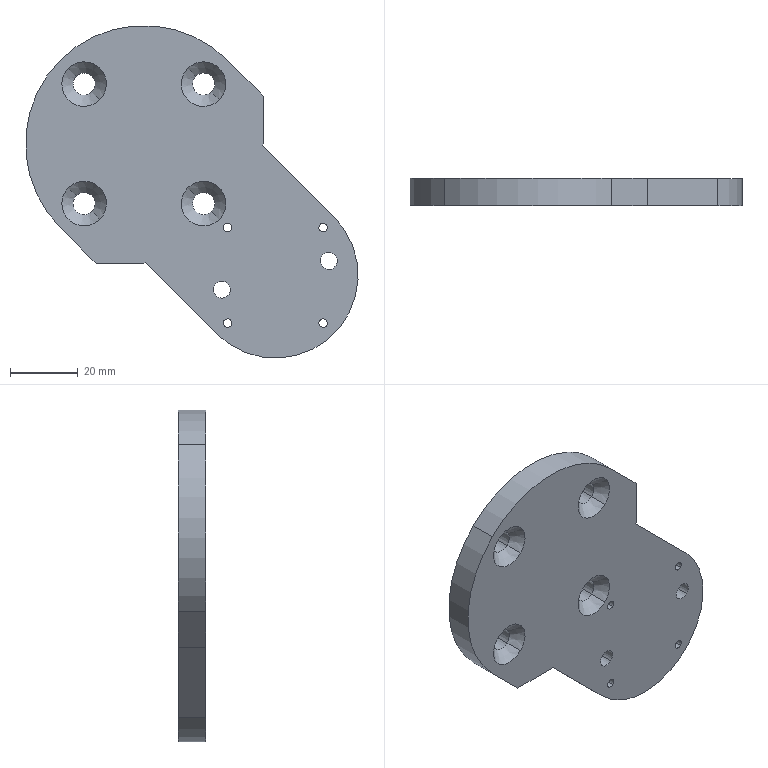Component | SolidWorks | F-SZP17248-10-11-1 | 1 solid | 41 faces | box 98.39 x 8 x 98.39 mm | volume 45727 mm3 | cylinder 23 | plane 10 | cone 8 | commonest cylinder face diameters 6.6 x8 2.5 x8 5.01 x4 70 x2 49 x1